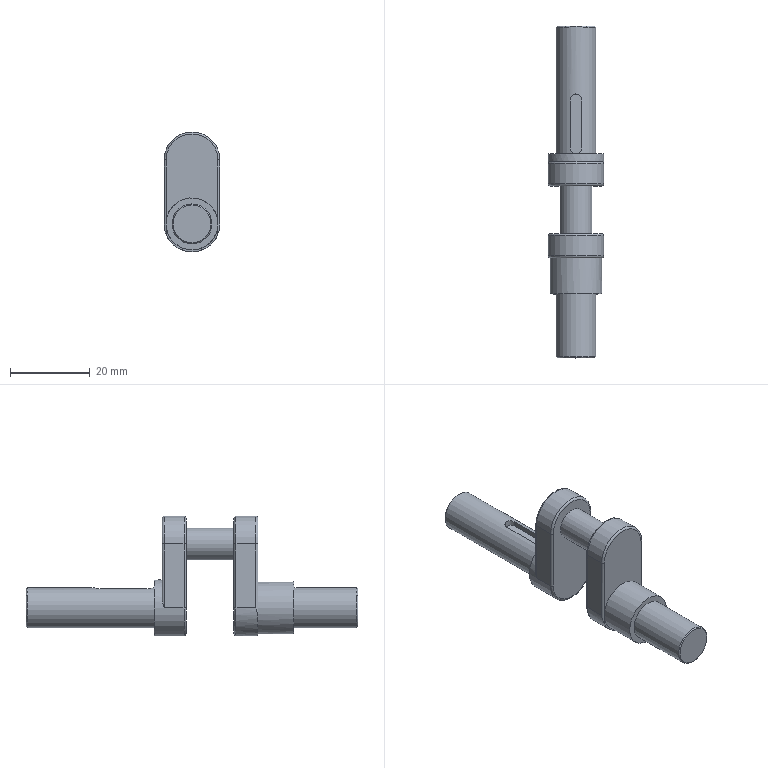Component | NX | CRANKSHAFT_2 | 1 solid | 42 faces | volume 10334 mm3 | cylinder 18 | plane 16 | torus 6 | cone 2 | commonest cylinder face diameters 1 x8 14 x4 10 x2 3 x2 8 x1 13 x1